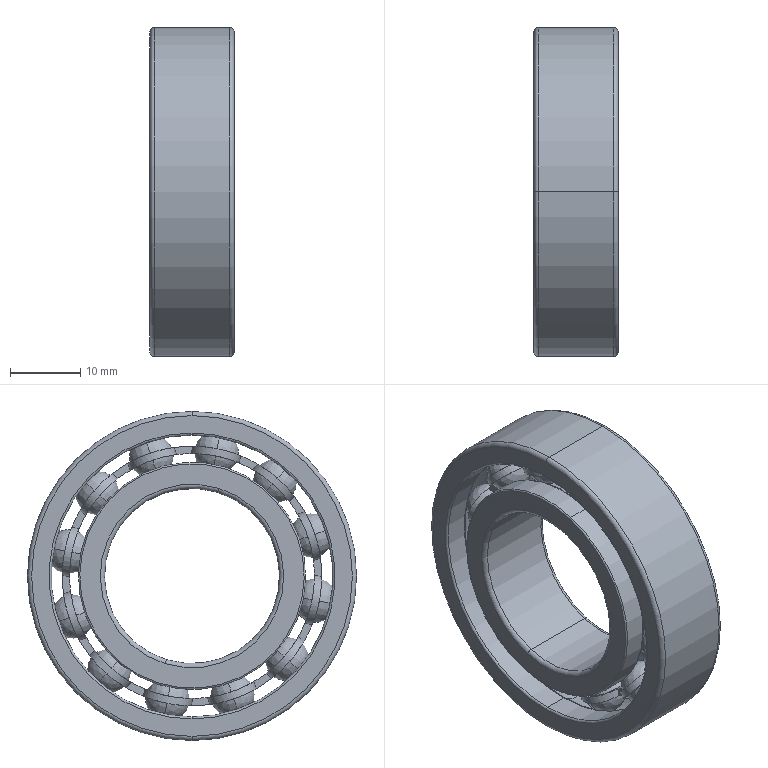Component | SolidWorks | 4-12-12ClampingAxisAssembly-1_4-12-4Bearing6005-2RZ-3 | 15 solids | 146 faces | volume 10323 mm3 | cylinder 64 | torus 30 | plane 28 | sphere 24 | commonest cylinder face diameters 6.277 x24 7.03 x24 40.231 x4 32.446 x4 47 x2 34.954 x2 37.046 x2 25 x2